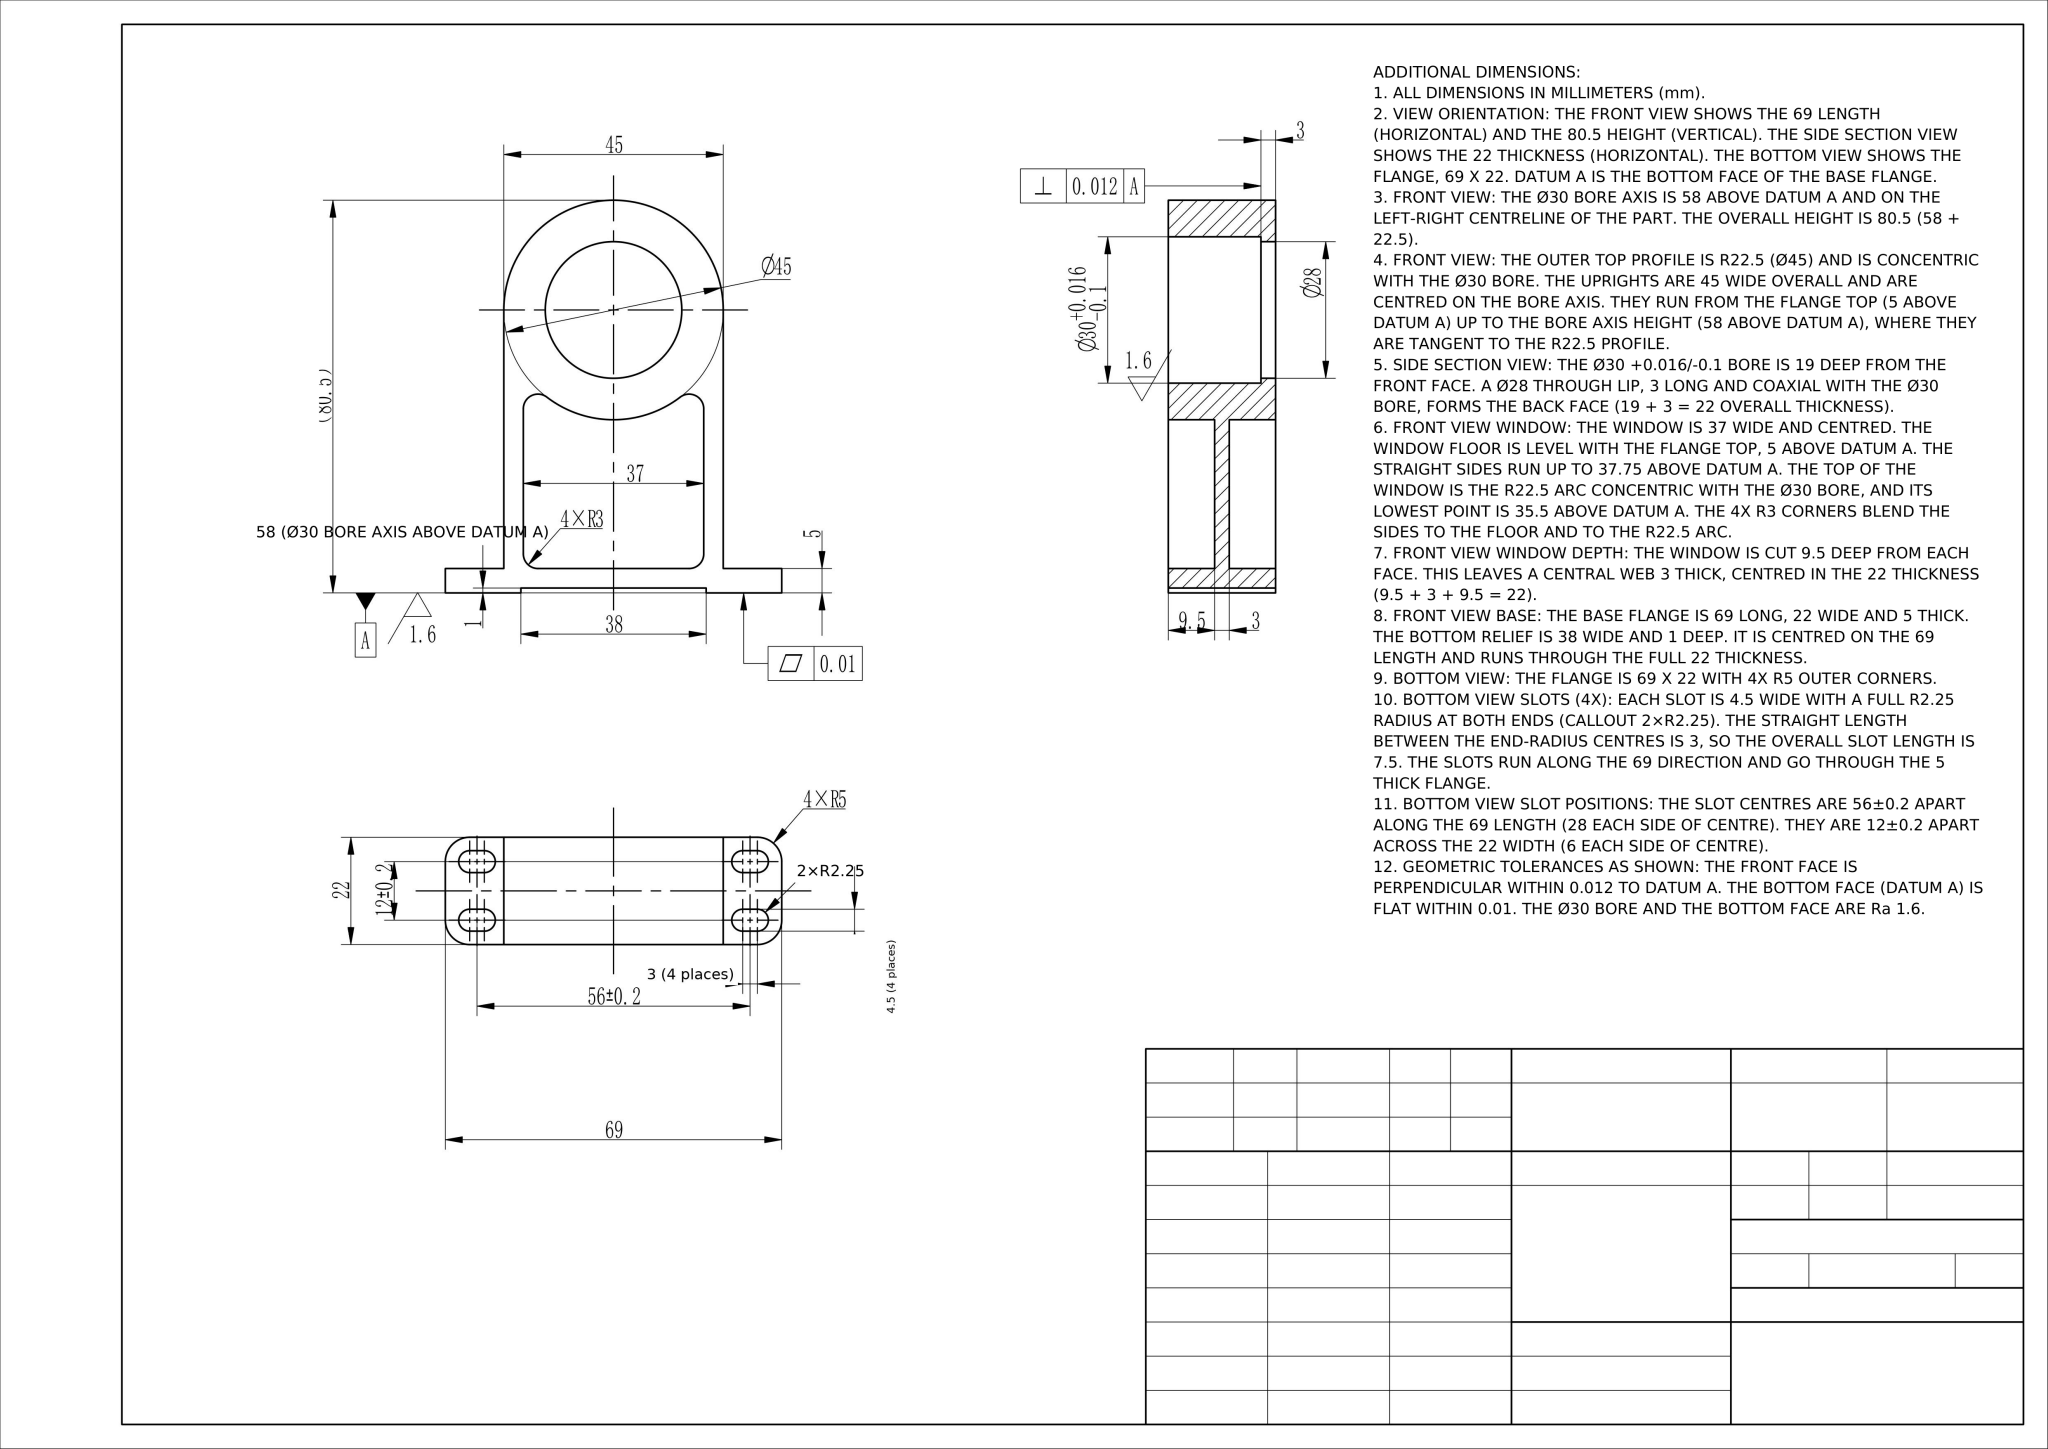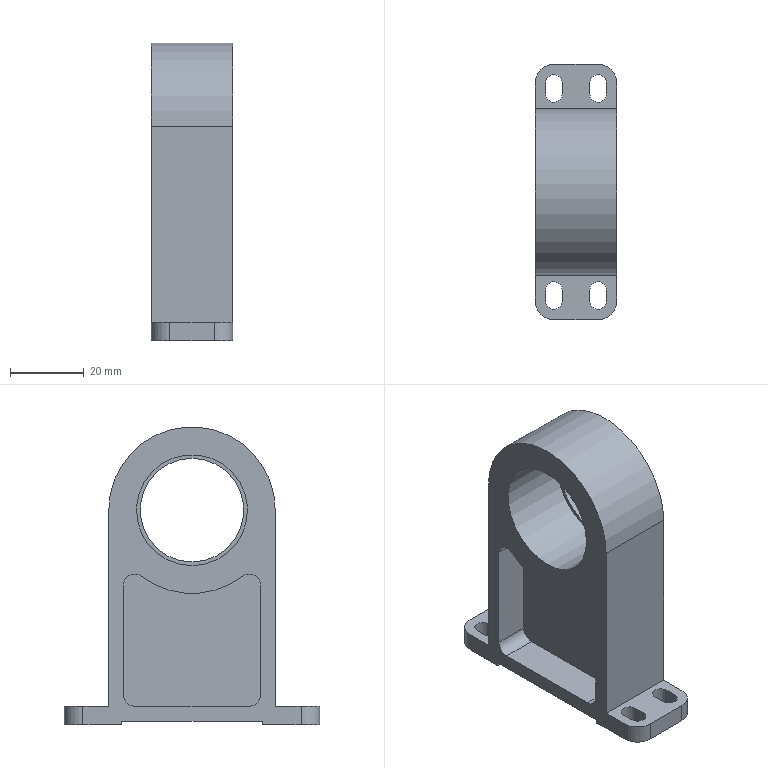Part | NX | mm | 1 solid | 55 faces | box 22 x 69 x 80.5 mm | volume 37736 mm3 | plane 30 | cylinder 25 | commonest cylinder face diameters 6 x8 4.5 x8 10 x4 45 x3 28 x1 30 x1